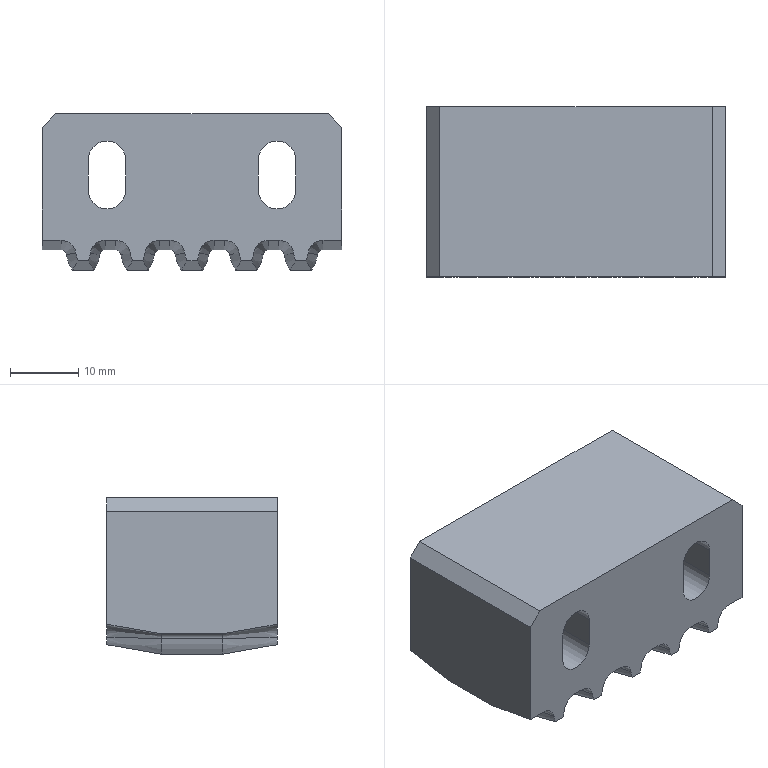Component | SolidWorks | SAWH02-03103A0SynchronousToothedMetalPart-1 | 1 solid | 118 faces | box 44 x 25 x 23 mm | volume 19626 mm3 | plane 50 | cone 40 | cylinder 28 | commonest cylinder face diameters 10.4 x10 1.6 x10 5.5 x4 10 x4 | material SUS304